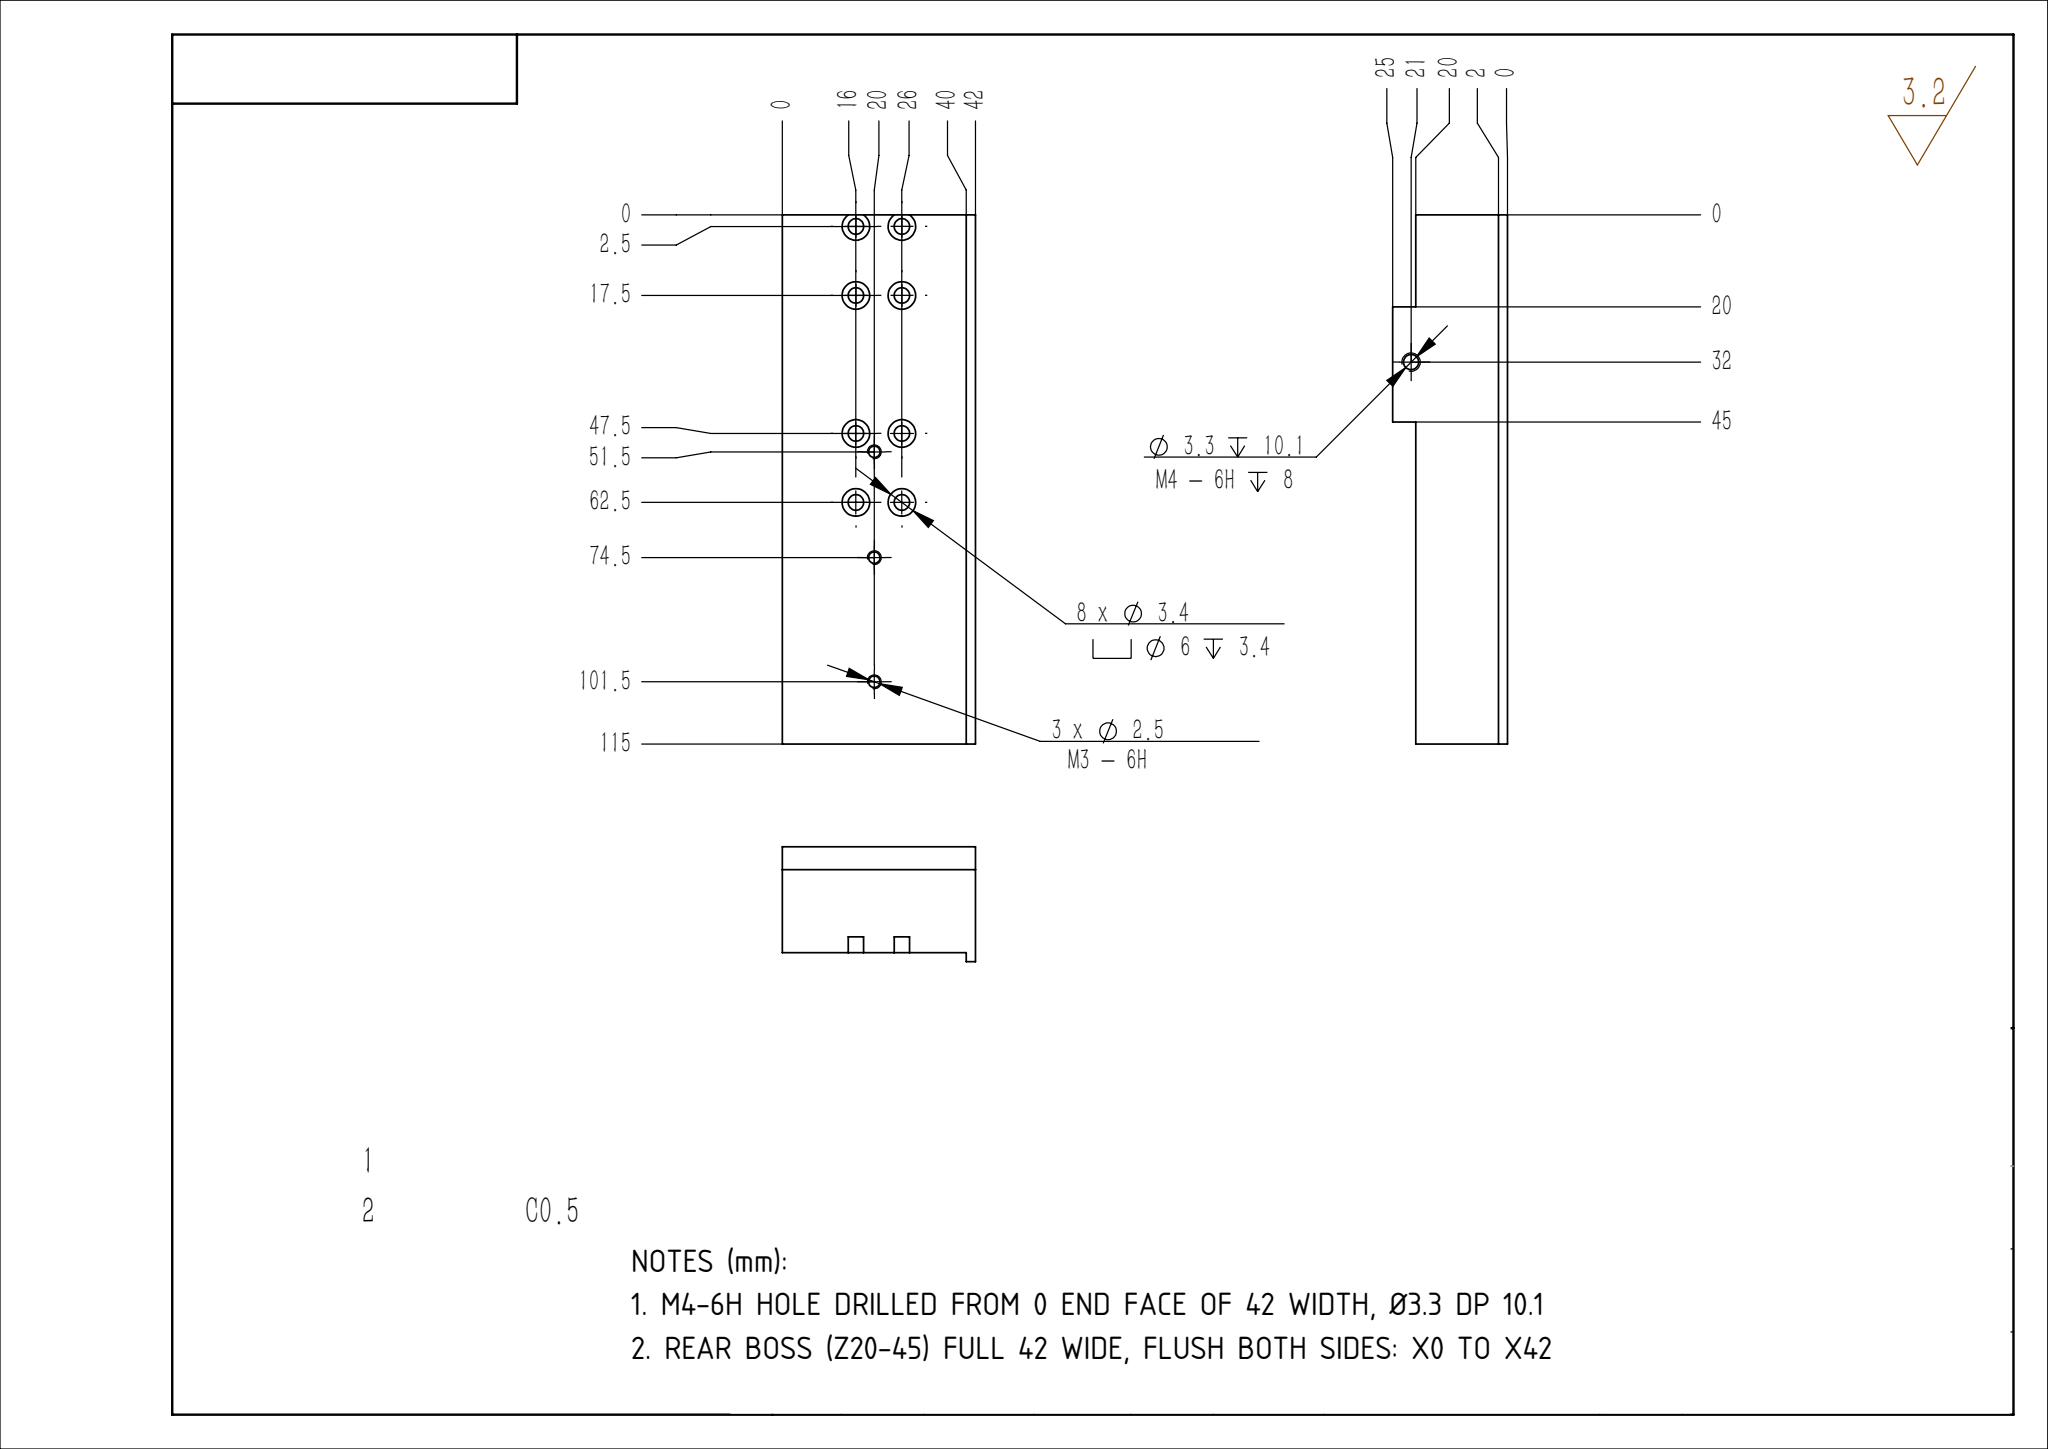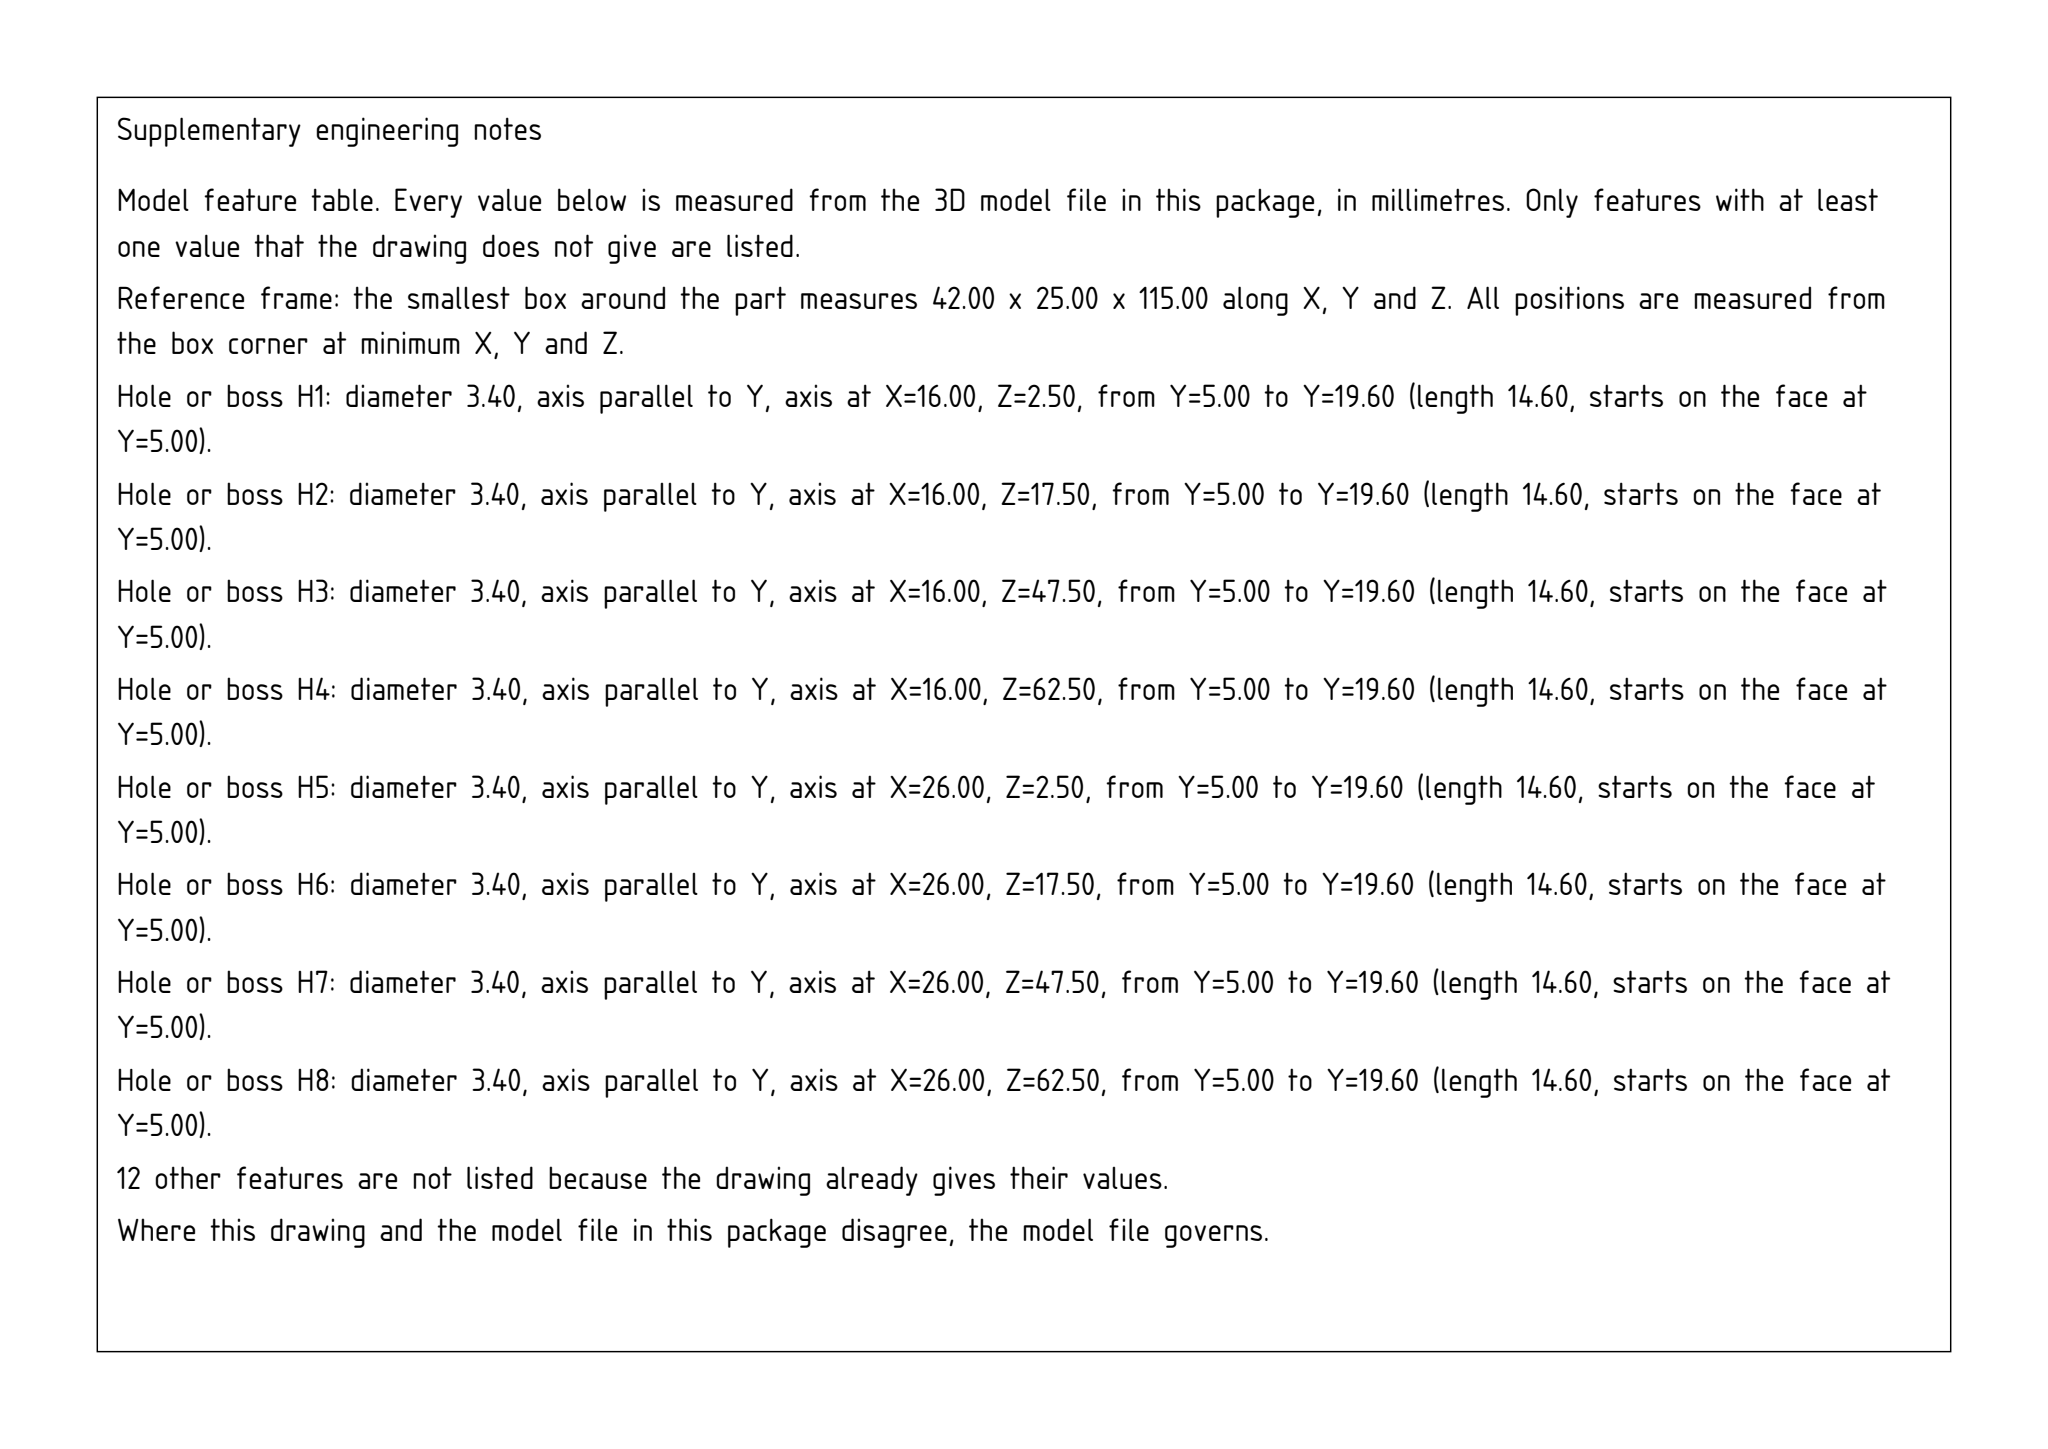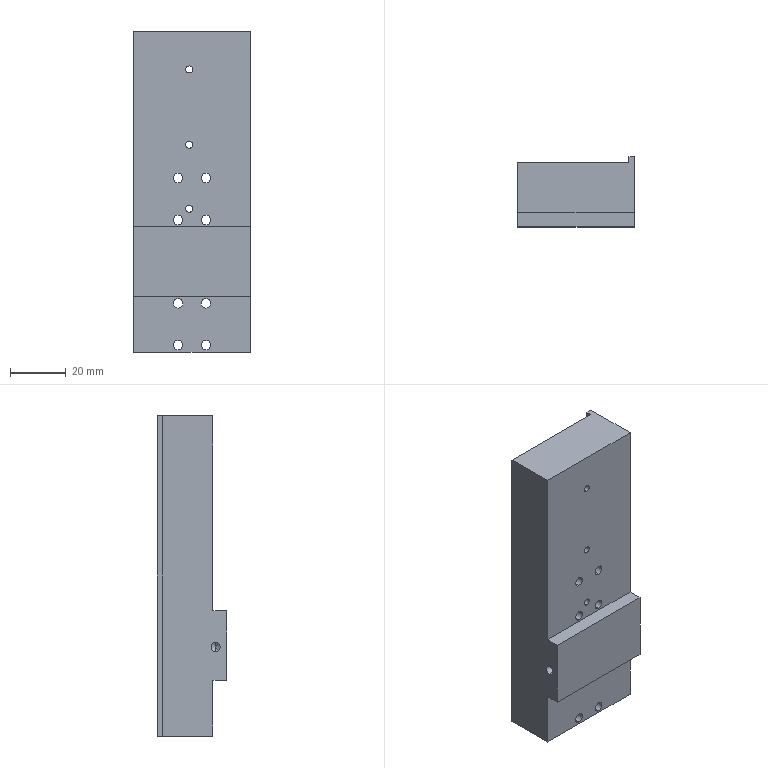Part | SolidWorks | mm | 1 solid | 62 faces | box 42 x 25 x 115 mm | volume 90474 mm3 | cylinder 40 | plane 20 | cone 2 | commonest cylinder face diameters 6 x16 3.4 x16 2.5 x6 3.3 x2
Drawing notes:
M4-6H HOLE DRILLED FROM 0 END FACE OF 42 WIDTH, Ø3.3 DP 10.1 | from the solid: Cylinder Ø3.3, axis X, at (y=4.0, z=32.0), length 10.1; X faces at 0/40/42; left view (normal X) shows hole open at x=0, so drill starts at x=0 end face
REAR BOSS (Z20-45) FULL 42 WIDE, FLUSH BOTH SIDES: X0 TO X42 | from the solid: Only x-planes 0/40/42; back face y=5 exists as 2 separate faces (z0-20 and z45-115), so boss spans full 42 width; M4 (Ø3.3↧10.1) holes enter from both x ends at y=4, z=32
build123d program:
from build123d import *

# Parameters (mm, degrees)
SKETCH1_W                                         = 42
SKETCH1_H                                         = 115
BOSS_EXTRUDE1_DEPTH                               = 18
SKETCH2_W                                         = 2
SKETCH2_H                                         = 115
BOSS_EXTRUDE2_DEPTH                               = 2
SKETCH3_W                                         = 42
SKETCH3_H                                         = 25
BOSS_EXTRUDE3_DEPTH                               = 5
M4_TAPPED_HOLE1_D                                 = 3.3
M4_TAPPED_HOLE1_DEPTH                             = 10.1
M4_TAPPED_HOLE1_TIP                               = 0.9914
HOLE_SIZE_ACCORDING_TO_HEXAGON_SOCKET_D           = 3.4
HOLE_SIZE_ACCORDING_TO_HEXAGON_SOCKET_CBORE_D     = 6
HOLE_SIZE_ACCORDING_TO_HEXAGON_SOCKET_CBORE_DEPTH = 3.4
LPATTERN2_COUNT                                   = 2
LPATTERN2_PITCH                                   = 45
M3_TAPPED_HOLE1_D                                 = 2.5


with BuildPart() as part:
    # Sketch1 → Boss-Extrude1 (new body)
    with BuildSketch(Plane(origin=(0, 0, 0), x_dir=(1, 0, 0), z_dir=(0, 1, 0))):
        Rectangle(SKETCH1_W, SKETCH1_H)
    extrude(amount=BOSS_EXTRUDE1_DEPTH)

    # Sketch2 → Boss-Extrude2 (add)
    with BuildSketch(Plane(origin=(0, 18, 0), x_dir=(1, 0, 0), z_dir=(0, 1, 0))):
        with Locations((20, 0)):
            Rectangle(SKETCH2_W, SKETCH2_H)
    extrude(amount=BOSS_EXTRUDE2_DEPTH)

    # Sketch3 → Boss-Extrude3 (add)
    with BuildSketch(Plane.XZ):
        with Locations((0, -25)):
            Rectangle(SKETCH3_W, SKETCH3_H)
    extrude(amount=BOSS_EXTRUDE3_DEPTH)

    # M4 Tapped Hole1
    with Locations(Plane.ZY.offset(21)):
        with Locations((-25.5, -1)):
            Hole(M4_TAPPED_HOLE1_D / 2, depth=M4_TAPPED_HOLE1_DEPTH)
            with Locations((0, 0, -(M4_TAPPED_HOLE1_DEPTH + M4_TAPPED_HOLE1_TIP / 2))):  # 118° drill point
                Cone(0, M4_TAPPED_HOLE1_D / 2, M4_TAPPED_HOLE1_TIP, mode=Mode.SUBTRACT)

    # Hole Size _ according to_ Hexagon Socket (through all)
    with Locations(Plane(origin=(0, 18, 0), x_dir=(1, 0, 0), z_dir=(0, 1, 0))):
        with Locations((-5, 55), (5, 55), (-5, 40), (5, 40)):
            hole_size_according_to_hexagon_socket = CounterBoreHole(HOLE_SIZE_ACCORDING_TO_HEXAGON_SOCKET_D / 2, HOLE_SIZE_ACCORDING_TO_HEXAGON_SOCKET_CBORE_D / 2, HOLE_SIZE_ACCORDING_TO_HEXAGON_SOCKET_CBORE_DEPTH)

    # LPattern2: Hole Size _ according to_ Hexagon Socket ×2
    with Locations(*[(0, 0, i * LPATTERN2_PITCH) for i in range(1, LPATTERN2_COUNT)]):
        add(hole_size_according_to_hexagon_socket, mode=Mode.SUBTRACT)

    # M3 Tapped Hole1 (through all)
    with Locations(Plane(origin=(0, 18, 0), x_dir=(1, 0, 0), z_dir=(0, 1, 0))):
        with Locations((-1, 6), (-1, -17), (-1, -44)):
            Hole(M3_TAPPED_HOLE1_D / 2)


solid = part.part